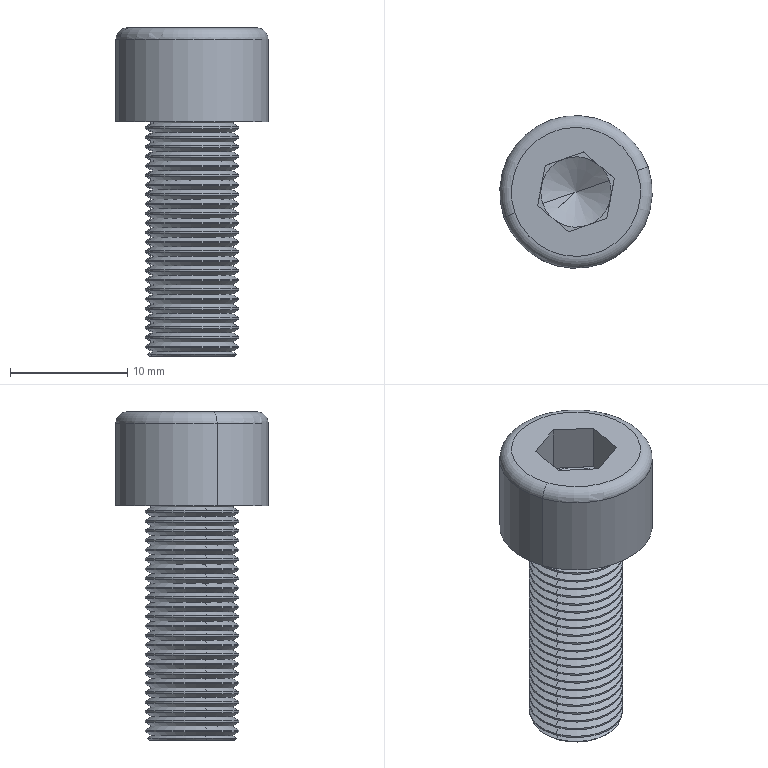Component | SolidWorks | HexagonSocketHeadCapScrew-M8X20-0510-1 | 1 solid | 174 faces | volume 1794 mm3 | cone 104 | cylinder 52 | plane 16 | torus 2 | commonest cylinder face diameters 8 x48 13 x2 9.353 x2